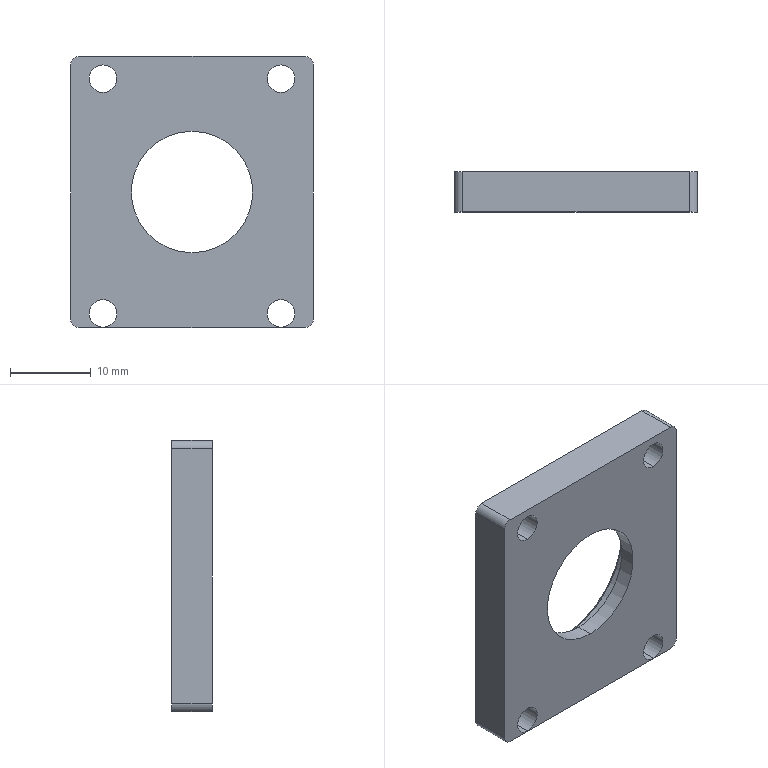Component | SolidWorks | FocusingLensHolder-1 | 1 solid | 25 faces | box 30 x 5 x 33.5 mm | volume 3535 mm3 | cylinder 16 | plane 7 | cone 2 | commonest cylinder face diameters 3.4 x8 2 x4 20 x2 15 x2
build123d program:
from build123d import *

# Parameters (mm, degrees)
SKETCH1_W           = 30
SKETCH1_H           = 33.5
SKETCH1_R           = 1.7
BOSS_EXTRUDE1_DEPTH = 5
SKETCH2_R           = 7.5
CUT_EXTRUDE1_DEPTH  = 6
SKETCH3_R           = 10
CUT_EXTRUDE2_DEPTH  = 3
CHAMFER1_SIZE       = 0.5
FILLET1_R           = 1


with BuildPart() as part:
    # Sketch1 → Boss-Extrude1 (new body)
    with BuildSketch(Plane(origin=(0, 0, 0), x_dir=(1, 0, 0), z_dir=(0, 1, 0))):
        Rectangle(SKETCH1_W, SKETCH1_H)
        with Locations(Location((-11, -14, 0), (0, 0, 270))):
            Circle(SKETCH1_R, mode=Mode.SUBTRACT)
        with Locations(Location((11, -14, 0), (0, 0, 90))):
            Circle(SKETCH1_R, mode=Mode.SUBTRACT)
        with Locations(Location((-11, 15, 0), (0, 0, 270))):
            Circle(SKETCH1_R, mode=Mode.SUBTRACT)
        with Locations(Location((11, 15, 0), (0, 0, 270))):
            Circle(SKETCH1_R, mode=Mode.SUBTRACT)
    extrude(amount=BOSS_EXTRUDE1_DEPTH)

    # Sketch2 → Cut-Extrude1 (cut)
    with BuildSketch(Plane(origin=(0, 5, 0), x_dir=(1, 0, 0), z_dir=(0, 1, 0))):
        with Locations(Location((0, 0, 0), (0, 0, 270))):
            Circle(SKETCH2_R)
    extrude(amount=-CUT_EXTRUDE1_DEPTH, mode=Mode.SUBTRACT)

    # Sketch3 → Cut-Extrude2 (cut)
    with BuildSketch(Plane(origin=(0, 5, 0), x_dir=(1, 0, 0), z_dir=(0, 1, 0))):
        with Locations(Location((0, 0, 0), (0, 0, 270))):
            Circle(SKETCH3_R)
    extrude(amount=-CUT_EXTRUDE2_DEPTH, mode=Mode.SUBTRACT)

    # Chamfer1
    chamfer1_edges = [part.edges().sort_by_distance(p)[0] for p in [
        (0, 5, -10),
    ]]
    chamfer(chamfer1_edges, length=CHAMFER1_SIZE)

    # Fillet1
    fillet1_edges = [part.edges().sort_by_distance(p)[0] for p in [
        (15, 2.5, 16.75),
        (-15, 2.5, 16.75),
        (-15, 2.5, -16.75),
        (15, 2.5, -16.75),
    ]]
    fillet(fillet1_edges, radius=FILLET1_R)


solid = part.part

# Placed as in the assembly
solid = solid.moved(Location((-5.981, 10.506, 205.812), (0, 0, 0)))
STEP:
#1=COLOUR_RGB('',0.7922,0.8196,0.9333);
#2=FILL_AREA_STYLE_COLOUR('',#1);
#3=FILL_AREA_STYLE('',(#2));
#4=SURFACE_STYLE_FILL_AREA(#3);
#5=SURFACE_SIDE_STYLE('',(#4));
#6=SURFACE_STYLE_USAGE(.BOTH.,#5);
#7=PRESENTATION_STYLE_ASSIGNMENT((#6));
#8=CARTESIAN_POINT('',(-0.2355,0.5908,7.709));
#9=VERTEX_POINT('',#8);
#10=CARTESIAN_POINT('',(-0.2355,0.5908,8.497));
#11=VERTEX_POINT('',#10);
#12=CARTESIAN_POINT('',(-0.2355,0.5908,8.103));
#13=DIRECTION('',(0.,1.,0.));
#14=DIRECTION('',(0.,0.,1.));
#15=AXIS2_PLACEMENT_3D('',#12,#13,#14);
#16=CIRCLE('',#15,0.3937);
#17=EDGE_CURVE('',#9,#11,#16,.T.);
#18=ORIENTED_EDGE('',*,*,#17,.F.);
#19=CARTESIAN_POINT('',(-0.2355,0.6105,7.689));
#20=VERTEX_POINT('',#19);
#21=CARTESIAN_POINT('',(-0.2355,0.5908,7.709));
#22=DIRECTION('',(0.,0.7071,-0.7071));
#23=VECTOR('',#22,39.37);
#24=LINE('',#21,#23);
#25=EDGE_CURVE('',#9,#20,#24,.T.);
#26=ORIENTED_EDGE('',*,*,#25,.T.);
#27=CARTESIAN_POINT('',(-0.2355,0.6105,8.516));
#28=VERTEX_POINT('',#27);
#29=CARTESIAN_POINT('',(-0.2355,0.6105,8.103));
#30=DIRECTION('',(0.,-1.,0.));
#31=DIRECTION('',(0.,0.,1.));
#32=AXIS2_PLACEMENT_3D('',#29,#30,#31);
#33=CIRCLE('',#32,0.4134);
#34=EDGE_CURVE('',#28,#20,#33,.T.);
#35=ORIENTED_EDGE('',*,*,#34,.F.);
#36=CARTESIAN_POINT('',(-0.2355,0.5908,8.497));
#37=DIRECTION('',(0.,0.7071,0.7071));
#38=VECTOR('',#37,39.37);
#39=LINE('',#36,#38);
#40=EDGE_CURVE('',#11,#28,#39,.T.);
#41=ORIENTED_EDGE('',*,*,#40,.F.);
#42=EDGE_LOOP('',(#18,#26,#35,#41));
#43=FACE_OUTER_BOUND('',#42,.T.);
#44=CARTESIAN_POINT('',(-0.2355,0.5908,8.103));
#45=DIRECTION('',(0.,1.,0.));
#46=DIRECTION('',(0.,0.,1.));
#47=AXIS2_PLACEMENT_3D('',#44,#45,#46);
#48=CONICAL_SURFACE('',#47,0.3937,0.7854);
#49=ADVANCED_FACE('',(#43),#48,.F.);
#50=CARTESIAN_POINT('',(-0.2355,0.4924,7.709));
#51=VERTEX_POINT('',#50);
#52=CARTESIAN_POINT('',(-0.2355,0.4924,8.497));
#53=VERTEX_POINT('',#52);
#54=CARTESIAN_POINT('',(-0.2355,0.4924,8.103));
#55=DIRECTION('',(0.,1.,0.));
#56=DIRECTION('',(0.,0.,1.));
#57=AXIS2_PLACEMENT_3D('',#54,#55,#56);
#58=CIRCLE('',#57,0.3937);
#59=EDGE_CURVE('',#51,#53,#58,.T.);
#60=ORIENTED_EDGE('',*,*,#59,.F.);
#61=CARTESIAN_POINT('',(-0.2355,0.4924,7.709));
#62=DIRECTION('',(0.,1.,0.));
#63=VECTOR('',#62,39.37);
#64=LINE('',#61,#63);
#65=EDGE_CURVE('',#51,#9,#64,.T.);
#66=ORIENTED_EDGE('',*,*,#65,.T.);
#67=ORIENTED_EDGE('',*,*,#17,.T.);
#68=CARTESIAN_POINT('',(-0.2355,0.4924,8.497));
#69=DIRECTION('',(0.,1.,0.));
#70=VECTOR('',#69,39.37);
#71=LINE('',#68,#70);
#72=EDGE_CURVE('',#53,#11,#71,.T.);
#73=ORIENTED_EDGE('',*,*,#72,.F.);
#74=EDGE_LOOP('',(#60,#66,#67,#73));
#75=FACE_OUTER_BOUND('',#74,.T.);
#76=CARTESIAN_POINT('',(-0.2355,0.4924,8.103));
#77=DIRECTION('',(0.,1.,0.));
#78=DIRECTION('',(0.,0.,1.));
#79=AXIS2_PLACEMENT_3D('',#76,#77,#78);
#80=CYLINDRICAL_SURFACE('',#79,0.3937);
#81=ADVANCED_FACE('',(#75),#80,.F.);
#82=CARTESIAN_POINT('',(0.1976,0.6105,7.445));
#83=VERTEX_POINT('',#82);
#84=CARTESIAN_POINT('',(0.1976,0.6105,7.579));
#85=VERTEX_POINT('',#84);
#86=CARTESIAN_POINT('',(0.1976,0.6105,7.512));
#87=DIRECTION('',(0.,1.,0.));
#88=DIRECTION('',(0.,0.,1.));
#89=AXIS2_PLACEMENT_3D('',#86,#87,#88);
#90=CIRCLE('',#89,0.06693);
#91=EDGE_CURVE('',#83,#85,#90,.T.);
#92=ORIENTED_EDGE('',*,*,#91,.T.);
#93=CARTESIAN_POINT('',(0.1976,0.4136,7.579));
#94=VERTEX_POINT('',#93);
#95=CARTESIAN_POINT('',(0.1976,0.6105,7.579));
#96=DIRECTION('',(0.,-1.,0.));
#97=VECTOR('',#96,39.37);
#98=LINE('',#95,#97);
#99=EDGE_CURVE('',#85,#94,#98,.T.);
#100=ORIENTED_EDGE('',*,*,#99,.T.);
#101=CARTESIAN_POINT('',(0.1976,0.4136,7.445));
#102=VERTEX_POINT('',#101);
#103=CARTESIAN_POINT('',(0.1976,0.4136,7.512));
#104=DIRECTION('',(0.,1.,0.));
#105=DIRECTION('',(0.,0.,1.));
#106=AXIS2_PLACEMENT_3D('',#103,#104,#105);
#107=CIRCLE('',#106,0.06693);
#108=EDGE_CURVE('',#102,#94,#107,.T.);
#109=ORIENTED_EDGE('',*,*,#108,.F.);
#110=CARTESIAN_POINT('',(0.1976,0.6105,7.445));
#111=DIRECTION('',(0.,-1.,0.));
#112=VECTOR('',#111,39.37);
#113=LINE('',#110,#112);
#114=EDGE_CURVE('',#83,#102,#113,.T.);
#115=ORIENTED_EDGE('',*,*,#114,.F.);
#116=EDGE_LOOP('',(#92,#100,#109,#115));
#117=FACE_OUTER_BOUND('',#116,.T.);
#118=CARTESIAN_POINT('',(0.1976,0.6105,7.512));
#119=DIRECTION('',(0.,-1.,0.));
#120=DIRECTION('',(0.,0.,-1.));
#121=AXIS2_PLACEMENT_3D('',#118,#119,#120);
#122=CYLINDRICAL_SURFACE('',#121,0.06693);
#123=ADVANCED_FACE('',(#117),#122,.F.);
#124=CARTESIAN_POINT('',(-0.6685,0.6105,7.445));
#125=VERTEX_POINT('',#124);
#126=CARTESIAN_POINT('',(-0.6685,0.6105,7.579));
#127=VERTEX_POINT('',#126);
#128=CARTESIAN_POINT('',(-0.6685,0.6105,7.512));
#129=DIRECTION('',(0.,1.,0.));
#130=DIRECTION('',(0.,0.,1.));
#131=AXIS2_PLACEMENT_3D('',#128,#129,#130);
#132=CIRCLE('',#131,0.06693);
#133=EDGE_CURVE('',#125,#127,#132,.T.);
#134=ORIENTED_EDGE('',*,*,#133,.T.);
#135=CARTESIAN_POINT('',(-0.6685,0.4136,7.579));
#136=VERTEX_POINT('',#135);
#137=CARTESIAN_POINT('',(-0.6685,0.6105,7.579));
#138=DIRECTION('',(0.,-1.,0.));
#139=VECTOR('',#138,39.37);
#140=LINE('',#137,#139);
#141=EDGE_CURVE('',#127,#136,#140,.T.);
#142=ORIENTED_EDGE('',*,*,#141,.T.);
#143=CARTESIAN_POINT('',(-0.6685,0.4136,7.445));
#144=VERTEX_POINT('',#143);
#145=CARTESIAN_POINT('',(-0.6685,0.4136,7.512));
#146=DIRECTION('',(0.,1.,0.));
#147=DIRECTION('',(0.,0.,1.));
#148=AXIS2_PLACEMENT_3D('',#145,#146,#147);
#149=CIRCLE('',#148,0.06693);
#150=EDGE_CURVE('',#144,#136,#149,.T.);
#151=ORIENTED_EDGE('',*,*,#150,.F.);
#152=CARTESIAN_POINT('',(-0.6685,0.6105,7.445));
#153=DIRECTION('',(0.,-1.,0.));
#154=VECTOR('',#153,39.37);
#155=LINE('',#152,#154);
#156=EDGE_CURVE('',#125,#144,#155,.T.);
#157=ORIENTED_EDGE('',*,*,#156,.F.);
#158=EDGE_LOOP('',(#134,#142,#151,#157));
#159=FACE_OUTER_BOUND('',#158,.T.);
#160=CARTESIAN_POINT('',(-0.6685,0.6105,7.512));
#161=DIRECTION('',(0.,-1.,0.));
#162=DIRECTION('',(0.,0.,-1.));
#163=AXIS2_PLACEMENT_3D('',#160,#161,#162);
#164=CYLINDRICAL_SURFACE('',#163,0.06693);
#165=ADVANCED_FACE('',(#159),#164,.F.);
#166=CARTESIAN_POINT('',(0.1976,0.6105,8.587));
#167=VERTEX_POINT('',#166);
#168=CARTESIAN_POINT('',(0.1976,0.6105,8.721));
#169=VERTEX_POINT('',#168);
#170=CARTESIAN_POINT('',(0.1976,0.6105,8.654));
#171=DIRECTION('',(0.,1.,0.));
#172=DIRECTION('',(0.,0.,-1.));
#173=AXIS2_PLACEMENT_3D('',#170,#171,#172);
#174=CIRCLE('',#173,0.06693);
#175=EDGE_CURVE('',#167,#169,#174,.T.);
#176=ORIENTED_EDGE('',*,*,#175,.T.);
#177=CARTESIAN_POINT('',(0.1976,0.4136,8.721));
#178=VERTEX_POINT('',#177);
#179=CARTESIAN_POINT('',(0.1976,0.6105,8.721));
#180=DIRECTION('',(0.,-1.,0.));
#181=VECTOR('',#180,39.37);
#182=LINE('',#179,#181);
#183=EDGE_CURVE('',#169,#178,#182,.T.);
#184=ORIENTED_EDGE('',*,*,#183,.T.);
#185=CARTESIAN_POINT('',(0.1976,0.4136,8.587));
#186=VERTEX_POINT('',#185);
#187=CARTESIAN_POINT('',(0.1976,0.4136,8.654));
#188=DIRECTION('',(0.,1.,0.));
#189=DIRECTION('',(0.,0.,-1.));
#190=AXIS2_PLACEMENT_3D('',#187,#188,#189);
#191=CIRCLE('',#190,0.06693);
#192=EDGE_CURVE('',#186,#178,#191,.T.);
#193=ORIENTED_EDGE('',*,*,#192,.F.);
#194=CARTESIAN_POINT('',(0.1976,0.6105,8.587));
#195=DIRECTION('',(0.,-1.,0.));
#196=VECTOR('',#195,39.37);
#197=LINE('',#194,#196);
#198=EDGE_CURVE('',#167,#186,#197,.T.);
#199=ORIENTED_EDGE('',*,*,#198,.F.);
#200=EDGE_LOOP('',(#176,#184,#193,#199));
#201=FACE_OUTER_BOUND('',#200,.T.);
#202=CARTESIAN_POINT('',(0.1976,0.6105,8.654));
#203=DIRECTION('',(0.,-1.,0.));
#204=DIRECTION('',(0.,0.,-1.));
#205=AXIS2_PLACEMENT_3D('',#202,#203,#204);
#206=CYLINDRICAL_SURFACE('',#205,0.06693);
#207=ADVANCED_FACE('',(#201),#206,.F.);
#208=CARTESIAN_POINT('',(-0.6685,0.6105,8.587));
#209=VERTEX_POINT('',#208);
#210=CARTESIAN_POINT('',(-0.6685,0.6105,8.721));
#211=VERTEX_POINT('',#210);
#212=CARTESIAN_POINT('',(-0.6685,0.6105,8.654));
#213=DIRECTION('',(0.,1.,0.));
#214=DIRECTION('',(0.,0.,1.));
#215=AXIS2_PLACEMENT_3D('',#212,#213,#214);
#216=CIRCLE('',#215,0.06693);
#217=EDGE_CURVE('',#209,#211,#216,.T.);
#218=ORIENTED_EDGE('',*,*,#217,.T.);
#219=CARTESIAN_POINT('',(-0.6685,0.4136,8.721));
#220=VERTEX_POINT('',#219);
#221=CARTESIAN_POINT('',(-0.6685,0.6105,8.721));
#222=DIRECTION('',(0.,-1.,0.));
#223=VECTOR('',#222,39.37);
#224=LINE('',#221,#223);
#225=EDGE_CURVE('',#211,#220,#224,.T.);
#226=ORIENTED_EDGE('',*,*,#225,.T.);
#227=CARTESIAN_POINT('',(-0.6685,0.4136,8.587));
#228=VERTEX_POINT('',#227);
#229=CARTESIAN_POINT('',(-0.6685,0.4136,8.654));
#230=DIRECTION('',(0.,1.,0.));
#231=DIRECTION('',(0.,0.,1.));
#232=AXIS2_PLACEMENT_3D('',#229,#230,#231);
#233=CIRCLE('',#232,0.06693);
#234=EDGE_CURVE('',#228,#220,#233,.T.);
#235=ORIENTED_EDGE('',*,*,#234,.F.);
#236=CARTESIAN_POINT('',(-0.6685,0.6105,8.587));
#237=DIRECTION('',(0.,-1.,0.));
#238=VECTOR('',#237,39.37);
#239=LINE('',#236,#238);
#240=EDGE_CURVE('',#209,#228,#239,.T.);
#241=ORIENTED_EDGE('',*,*,#240,.F.);
#242=EDGE_LOOP('',(#218,#226,#235,#241));
#243=FACE_OUTER_BOUND('',#242,.T.);
#244=CARTESIAN_POINT('',(-0.6685,0.6105,8.654));
#245=DIRECTION('',(0.,-1.,0.));
#246=DIRECTION('',(0.,0.,-1.));
#247=AXIS2_PLACEMENT_3D('',#244,#245,#246);
#248=CYLINDRICAL_SURFACE('',#247,0.06693);
#249=ADVANCED_FACE('',(#243),#248,.F.);
#250=CARTESIAN_POINT('',(-0.2355,0.4136,7.808));
#251=VERTEX_POINT('',#250);
#252=CARTESIAN_POINT('',(-0.2355,0.4136,8.398));
#253=VERTEX_POINT('',#252);
#254=CARTESIAN_POINT('',(-0.2355,0.4136,8.103));
#255=DIRECTION('',(0.,1.,0.));
#256=DIRECTION('',(0.,0.,1.));
#257=AXIS2_PLACEMENT_3D('',#254,#255,#256);
#258=CIRCLE('',#257,0.2953);
#259=EDGE_CURVE('',#251,#253,#258,.T.);
#260=ORIENTED_EDGE('',*,*,#259,.F.);
#261=CARTESIAN_POINT('',(-0.2355,0.4924,7.808));
#262=VERTEX_POINT('',#261);
#263=CARTESIAN_POINT('',(-0.2355,0.3743,7.808));
#264=DIRECTION('',(0.,1.,0.));
#265=VECTOR('',#264,39.37);
#266=LINE('',#263,#265);
#267=EDGE_CURVE('',#251,#262,#266,.T.);
#268=ORIENTED_EDGE('',*,*,#267,.T.);
#269=CARTESIAN_POINT('',(-0.2355,0.4924,8.398));
#270=VERTEX_POINT('',#269);
#271=CARTESIAN_POINT('',(-0.2355,0.4924,8.103));
#272=DIRECTION('',(0.,-1.,0.));
#273=DIRECTION('',(0.,0.,1.));
#274=AXIS2_PLACEMENT_3D('',#271,#272,#273);
#275=CIRCLE('',#274,0.2953);
#276=EDGE_CURVE('',#270,#262,#275,.T.);
#277=ORIENTED_EDGE('',*,*,#276,.F.);
#278=CARTESIAN_POINT('',(-0.2355,0.3743,8.398));
#279=DIRECTION('',(0.,1.,0.));
#280=VECTOR('',#279,39.37);
#281=LINE('',#278,#280);
#282=EDGE_CURVE('',#253,#270,#281,.T.);
#283=ORIENTED_EDGE('',*,*,#282,.F.);
#284=EDGE_LOOP('',(#260,#268,#277,#283));
#285=FACE_OUTER_BOUND('',#284,.T.);
#286=CARTESIAN_POINT('',(-0.2355,0.3743,8.103));
#287=DIRECTION('',(0.,1.,0.));
#288=DIRECTION('',(0.,0.,1.));
#289=AXIS2_PLACEMENT_3D('',#286,#287,#288);
#290=CYLINDRICAL_SURFACE('',#289,0.2953);
#291=ADVANCED_FACE('',(#285),#290,.F.);
#292=ORIENTED_EDGE('',*,*,#267,.F.);
#293=CARTESIAN_POINT('',(-0.2355,0.4136,8.103));
#294=DIRECTION('',(0.,1.,0.));
#295=DIRECTION('',(0.,0.,1.));
#296=AXIS2_PLACEMENT_3D('',#293,#294,#295);
#297=CIRCLE('',#296,0.2953);
#298=EDGE_CURVE('',#253,#251,#297,.T.);
#299=ORIENTED_EDGE('',*,*,#298,.F.);
#300=ORIENTED_EDGE('',*,*,#282,.T.);
#301=CARTESIAN_POINT('',(-0.2355,0.4924,8.103));
#302=DIRECTION('',(0.,-1.,0.));
#303=DIRECTION('',(0.,0.,1.));
#304=AXIS2_PLACEMENT_3D('',#301,#302,#303);
#305=CIRCLE('',#304,0.2953);
#306=EDGE_CURVE('',#262,#270,#305,.T.);
#307=ORIENTED_EDGE('',*,*,#306,.F.);
#308=EDGE_LOOP('',(#292,#299,#300,#307));
#309=FACE_OUTER_BOUND('',#308,.T.);
#310=CARTESIAN_POINT('',(-0.2355,0.3743,8.103));
#311=DIRECTION('',(0.,1.,0.));
#312=DIRECTION('',(0.,0.,1.));
#313=AXIS2_PLACEMENT_3D('',#310,#311,#312);
#314=CYLINDRICAL_SURFACE('',#313,0.2953);
#315=ADVANCED_FACE('',(#309),#314,.F.);
#316=ORIENTED_EDGE('',*,*,#34,.T.);
#317=CARTESIAN_POINT('',(-0.2355,0.6105,8.103));
#318=DIRECTION('',(0.,-1.,0.));
#319=DIRECTION('',(0.,0.,1.));
#320=AXIS2_PLACEMENT_3D('',#317,#318,#319);
#321=CIRCLE('',#320,0.4134);
#322=EDGE_CURVE('',#20,#28,#321,.T.);
#323=ORIENTED_EDGE('',*,*,#322,.T.);
#324=EDGE_LOOP('',(#316,#323));
#325=FACE_BOUND('',#324,.T.);
#326=ORIENTED_EDGE('',*,*,#133,.F.);
#327=CARTESIAN_POINT('',(-0.6685,0.6105,7.512));
#328=DIRECTION('',(0.,1.,0.));
#329=DIRECTION('',(0.,0.,1.));
#330=AXIS2_PLACEMENT_3D('',#327,#328,#329);
#331=CIRCLE('',#330,0.06693);
#332=EDGE_CURVE('',#127,#125,#331,.T.);
#333=ORIENTED_EDGE('',*,*,#332,.F.);
#334=EDGE_LOOP('',(#326,#333));
#335=FACE_BOUND('',#334,.T.);
#336=ORIENTED_EDGE('',*,*,#217,.F.);
#337=CARTESIAN_POINT('',(-0.6685,0.6105,8.654));
#338=DIRECTION('',(0.,1.,0.));
#339=DIRECTION('',(0.,0.,1.));
#340=AXIS2_PLACEMENT_3D('',#337,#338,#339);
#341=CIRCLE('',#340,0.06693);
#342=EDGE_CURVE('',#211,#209,#341,.T.);
#343=ORIENTED_EDGE('',*,*,#342,.F.);
#344=EDGE_LOOP('',(#336,#343));
#345=FACE_BOUND('',#344,.T.);
#346=CARTESIAN_POINT('',(-0.826,0.6105,7.483));
#347=VERTEX_POINT('',#346);
#348=CARTESIAN_POINT('',(-0.826,0.6105,8.723));
#349=VERTEX_POINT('',#348);
#350=CARTESIAN_POINT('',(-0.826,0.6105,7.443));
#351=DIRECTION('',(-0.,0.,1.));
#352=VECTOR('',#351,39.37);
#353=LINE('',#350,#352);
#354=EDGE_CURVE('',#347,#349,#353,.T.);
#355=ORIENTED_EDGE('',*,*,#354,.T.);
#356=CARTESIAN_POINT('',(-0.7866,0.6105,8.762));
#357=VERTEX_POINT('',#356);
#358=CARTESIAN_POINT('',(-0.7866,0.6105,8.723));
#359=DIRECTION('',(0.,1.,0.));
#360=DIRECTION('',(0.,0.,1.));
#361=AXIS2_PLACEMENT_3D('',#358,#359,#360);
#362=CIRCLE('',#361,0.03937);
#363=EDGE_CURVE('',#349,#357,#362,.T.);
#364=ORIENTED_EDGE('',*,*,#363,.T.);
#365=CARTESIAN_POINT('',(0.3157,0.6105,8.762));
#366=VERTEX_POINT('',#365);
#367=CARTESIAN_POINT('',(-0.826,0.6105,8.762));
#368=DIRECTION('',(1.,0.,0.));
#369=VECTOR('',#368,39.37);
#370=LINE('',#367,#369);
#371=EDGE_CURVE('',#357,#366,#370,.T.);
#372=ORIENTED_EDGE('',*,*,#371,.T.);
#373=CARTESIAN_POINT('',(0.3551,0.6105,8.723));
#374=VERTEX_POINT('',#373);
#375=CARTESIAN_POINT('',(0.3157,0.6105,8.723));
#376=DIRECTION('',(0.,1.,0.));
#377=DIRECTION('',(0.,0.,1.));
#378=AXIS2_PLACEMENT_3D('',#375,#376,#377);
#379=CIRCLE('',#378,0.03937);
#380=EDGE_CURVE('',#366,#374,#379,.T.);
#381=ORIENTED_EDGE('',*,*,#380,.T.);
#382=CARTESIAN_POINT('',(0.3551,0.6105,7.483));
#383=VERTEX_POINT('',#382);
#384=CARTESIAN_POINT('',(0.3551,0.6105,7.443));
#385=DIRECTION('',(0.,0.,-1.));
#386=VECTOR('',#385,39.37);
#387=LINE('',#384,#386);
#388=EDGE_CURVE('',#374,#383,#387,.T.);
#389=ORIENTED_EDGE('',*,*,#388,.T.);
#390=CARTESIAN_POINT('',(0.3157,0.6105,7.443));
#391=VERTEX_POINT('',#390);
#392=CARTESIAN_POINT('',(0.3157,0.6105,7.483));
#393=DIRECTION('',(0.,1.,0.));
#394=DIRECTION('',(0.,0.,1.));
#395=AXIS2_PLACEMENT_3D('',#392,#393,#394);
#396=CIRCLE('',#395,0.03937);
#397=EDGE_CURVE('',#383,#391,#396,.T.);
#398=ORIENTED_EDGE('',*,*,#397,.T.);
#399=CARTESIAN_POINT('',(-0.7866,0.6105,7.443));
#400=VERTEX_POINT('',#399);
#401=CARTESIAN_POINT('',(-0.826,0.6105,7.443));
#402=DIRECTION('',(-1.,0.,-0.));
#403=VECTOR('',#402,39.37);
#404=LINE('',#401,#403);
#405=EDGE_CURVE('',#391,#400,#404,.T.);
#406=ORIENTED_EDGE('',*,*,#405,.T.);
#407=CARTESIAN_POINT('',(-0.7866,0.6105,7.483));
#408=DIRECTION('',(0.,1.,0.));
#409=DIRECTION('',(0.,0.,1.));
#410=AXIS2_PLACEMENT_3D('',#407,#408,#409);
#411=CIRCLE('',#410,0.03937);
#412=EDGE_CURVE('',#400,#347,#411,.T.);
#413=ORIENTED_EDGE('',*,*,#412,.T.);
#414=EDGE_LOOP('',(#355,#364,#372,#381,#389,#398,#406,#413));
#415=FACE_OUTER_BOUND('',#414,.T.);
#416=ORIENTED_EDGE('',*,*,#175,.F.);
#417=CARTESIAN_POINT('',(0.1976,0.6105,8.654));
#418=DIRECTION('',(0.,1.,0.));
#419=DIRECTION('',(0.,0.,-1.));
#420=AXIS2_PLACEMENT_3D('',#417,#418,#419);
#421=CIRCLE('',#420,0.06693);
#422=EDGE_CURVE('',#169,#167,#421,.T.);
#423=ORIENTED_EDGE('',*,*,#422,.F.);
#424=EDGE_LOOP('',(#416,#423));
#425=FACE_BOUND('',#424,.T.);
#426=ORIENTED_EDGE('',*,*,#91,.F.);
#427=CARTESIAN_POINT('',(0.1976,0.6105,7.512));
#428=DIRECTION('',(0.,1.,0.));
#429=DIRECTION('',(0.,0.,1.));
#430=AXIS2_PLACEMENT_3D('',#427,#428,#429);
#431=CIRCLE('',#430,0.06693);
#432=EDGE_CURVE('',#85,#83,#431,.T.);
#433=ORIENTED_EDGE('',*,*,#432,.F.);
#434=EDGE_LOOP('',(#426,#433));
#435=FACE_BOUND('',#434,.T.);
#436=CARTESIAN_POINT('',(-0.2355,0.6105,8.103));
#437=DIRECTION('',(0.,1.,0.));
#438=DIRECTION('',(0.,0.,1.));
#439=AXIS2_PLACEMENT_3D('',#436,#437,#438);
#440=PLANE('',#439);
#441=ADVANCED_FACE('',(#325,#335,#345,#415,#425,#435),#440,.T.);
#442=ORIENTED_EDGE('',*,*,#298,.T.);
#443=ORIENTED_EDGE('',*,*,#259,.T.);
#444=EDGE_LOOP('',(#442,#443));
#445=FACE_BOUND('',#444,.T.);
#446=CARTESIAN_POINT('',(-0.7866,0.4136,8.762));
#447=VERTEX_POINT('',#446);
#448=CARTESIAN_POINT('',(0.3157,0.4136,8.762));
#449=VERTEX_POINT('',#448);
#450=CARTESIAN_POINT('',(-0.826,0.4136,8.762));
#451=DIRECTION('',(1.,0.,0.));
#452=VECTOR('',#451,39.37);
#453=LINE('',#450,#452);
#454=EDGE_CURVE('',#447,#449,#453,.T.);
#455=ORIENTED_EDGE('',*,*,#454,.F.);
#456=CARTESIAN_POINT('',(-0.826,0.4136,8.723));
#457=VERTEX_POINT('',#456);
#458=CARTESIAN_POINT('',(-0.7866,0.4136,8.723));
#459=DIRECTION('',(0.,-1.,0.));
#460=DIRECTION('',(0.,0.,1.));
#461=AXIS2_PLACEMENT_3D('',#458,#459,#460);
#462=CIRCLE('',#461,0.03937);
#463=EDGE_CURVE('',#447,#457,#462,.T.);
#464=ORIENTED_EDGE('',*,*,#463,.T.);
#465=CARTESIAN_POINT('',(-0.826,0.4136,7.483));
#466=VERTEX_POINT('',#465);
#467=CARTESIAN_POINT('',(-0.826,0.4136,7.443));
#468=DIRECTION('',(-0.,0.,1.));
#469=VECTOR('',#468,39.37);
#470=LINE('',#467,#469);
#471=EDGE_CURVE('',#466,#457,#470,.T.);
#472=ORIENTED_EDGE('',*,*,#471,.F.);
#473=CARTESIAN_POINT('',(-0.7866,0.4136,7.443));
#474=VERTEX_POINT('',#473);
#475=CARTESIAN_POINT('',(-0.7866,0.4136,7.483));
#476=DIRECTION('',(0.,-1.,0.));
#477=DIRECTION('',(0.,0.,1.));
#478=AXIS2_PLACEMENT_3D('',#475,#476,#477);
#479=CIRCLE('',#478,0.03937);
#480=EDGE_CURVE('',#466,#474,#479,.T.);
#481=ORIENTED_EDGE('',*,*,#480,.T.);
#482=CARTESIAN_POINT('',(0.3157,0.4136,7.443));
#483=VERTEX_POINT('',#482);
#484=CARTESIAN_POINT('',(-0.826,0.4136,7.443));
#485=DIRECTION('',(-1.,0.,-0.));
#486=VECTOR('',#485,39.37);
#487=LINE('',#484,#486);
#488=EDGE_CURVE('',#483,#474,#487,.T.);
#489=ORIENTED_EDGE('',*,*,#488,.F.);
#490=CARTESIAN_POINT('',(0.3551,0.4136,7.483));
#491=VERTEX_POINT('',#490);
#492=CARTESIAN_POINT('',(0.3157,0.4136,7.483));
#493=DIRECTION('',(0.,-1.,0.));
#494=DIRECTION('',(0.,0.,1.));
#495=AXIS2_PLACEMENT_3D('',#492,#493,#494);
#496=CIRCLE('',#495,0.03937);
#497=EDGE_CURVE('',#483,#491,#496,.T.);
#498=ORIENTED_EDGE('',*,*,#497,.T.);
#499=CARTESIAN_POINT('',(0.3551,0.4136,8.723));
#500=VERTEX_POINT('',#499);
#501=CARTESIAN_POINT('',(0.3551,0.4136,7.443));
#502=DIRECTION('',(0.,0.,-1.));
#503=VECTOR('',#502,39.37);
#504=LINE('',#501,#503);
#505=EDGE_CURVE('',#500,#491,#504,.T.);
#506=ORIENTED_EDGE('',*,*,#505,.F.);
#507=CARTESIAN_POINT('',(0.3157,0.4136,8.723));
#508=DIRECTION('',(0.,-1.,0.));
#509=DIRECTION('',(0.,0.,1.));
#510=AXIS2_PLACEMENT_3D('',#507,#508,#509);
#511=CIRCLE('',#510,0.03937);
#512=EDGE_CURVE('',#500,#449,#511,.T.);
#513=ORIENTED_EDGE('',*,*,#512,.T.);
#514=EDGE_LOOP('',(#455,#464,#472,#481,#489,#498,#506,#513));
#515=FACE_OUTER_BOUND('',#514,.T.);
#516=ORIENTED_EDGE('',*,*,#234,.T.);
#517=CARTESIAN_POINT('',(-0.6685,0.4136,8.654));
#518=DIRECTION('',(0.,1.,0.));
#519=DIRECTION('',(0.,0.,1.));
#520=AXIS2_PLACEMENT_3D('',#517,#518,#519);
#521=CIRCLE('',#520,0.06693);
#522=EDGE_CURVE('',#220,#228,#521,.T.);
#523=ORIENTED_EDGE('',*,*,#522,.T.);
#524=EDGE_LOOP('',(#516,#523));
#525=FACE_BOUND('',#524,.T.);
#526=ORIENTED_EDGE('',*,*,#192,.T.);
#527=CARTESIAN_POINT('',(0.1976,0.4136,8.654));
#528=DIRECTION('',(0.,1.,0.));
#529=DIRECTION('',(0.,0.,-1.));
#530=AXIS2_PLACEMENT_3D('',#527,#528,#529);
#531=CIRCLE('',#530,0.06693);
#532=EDGE_CURVE('',#178,#186,#531,.T.);
#533=ORIENTED_EDGE('',*,*,#532,.T.);
#534=EDGE_LOOP('',(#526,#533));
#535=FACE_BOUND('',#534,.T.);
#536=ORIENTED_EDGE('',*,*,#150,.T.);
#537=CARTESIAN_POINT('',(-0.6685,0.4136,7.512));
#538=DIRECTION('',(0.,1.,0.));
#539=DIRECTION('',(0.,0.,1.));
#540=AXIS2_PLACEMENT_3D('',#537,#538,#539);
#541=CIRCLE('',#540,0.06693);
#542=EDGE_CURVE('',#136,#144,#541,.T.);
#543=ORIENTED_EDGE('',*,*,#542,.T.);
#544=EDGE_LOOP('',(#536,#543));
#545=FACE_BOUND('',#544,.T.);
#546=ORIENTED_EDGE('',*,*,#108,.T.);
#547=CARTESIAN_POINT('',(0.1976,0.4136,7.512));
#548=DIRECTION('',(0.,1.,0.));
#549=DIRECTION('',(0.,0.,1.));
#550=AXIS2_PLACEMENT_3D('',#547,#548,#549);
#551=CIRCLE('',#550,0.06693);
#552=EDGE_CURVE('',#94,#102,#551,.T.);
#553=ORIENTED_EDGE('',*,*,#552,.T.);
#554=EDGE_LOOP('',(#546,#553));
#555=FACE_BOUND('',#554,.T.);
#556=CARTESIAN_POINT('',(-0.2355,0.4136,8.103));
#557=DIRECTION('',(0.,1.,0.));
#558=DIRECTION('',(0.,0.,1.));
#559=AXIS2_PLACEMENT_3D('',#556,#557,#558);
#560=PLANE('',#559);
#561=ADVANCED_FACE('',(#445,#515,#525,#535,#545,#555),#560,.F.);
#562=ORIENTED_EDGE('',*,*,#505,.T.);
#563=CARTESIAN_POINT('',(0.3551,0.6105,7.483));
#564=DIRECTION('',(0.,1.,0.));
#565=VECTOR('',#564,39.37);
#566=LINE('',#563,#565);
#567=EDGE_CURVE('',#491,#383,#566,.T.);
#568=ORIENTED_EDGE('',*,*,#567,.T.);
#569=ORIENTED_EDGE('',*,*,#388,.F.);
#570=CARTESIAN_POINT('',(0.3551,0.6105,8.723));
#571=DIRECTION('',(0.,-1.,0.));
#572=VECTOR('',#571,39.37);
#573=LINE('',#570,#572);
#574=EDGE_CURVE('',#374,#500,#573,.T.);
#575=ORIENTED_EDGE('',*,*,#574,.T.);
#576=EDGE_LOOP('',(#562,#568,#569,#575));
#577=FACE_OUTER_BOUND('',#576,.T.);
#578=CARTESIAN_POINT('',(0.3551,0.6105,7.443));
#579=DIRECTION('',(-1.,0.,-0.));
#580=DIRECTION('',(-0.,0.,1.));
#581=AXIS2_PLACEMENT_3D('',#578,#579,#580);
#582=PLANE('',#581);
#583=ADVANCED_FACE('',(#577),#582,.F.);
#584=ORIENTED_EDGE('',*,*,#488,.T.);
#585=CARTESIAN_POINT('',(-0.7866,0.6105,7.443));
#586=DIRECTION('',(0.,1.,0.));
#587=VECTOR('',#586,39.37);
#588=LINE('',#585,#587);
#589=EDGE_CURVE('',#474,#400,#588,.T.);
#590=ORIENTED_EDGE('',*,*,#589,.T.);
#591=ORIENTED_EDGE('',*,*,#405,.F.);
#592=CARTESIAN_POINT('',(0.3157,0.6105,7.443));
#593=DIRECTION('',(0.,-1.,0.));
#594=VECTOR('',#593,39.37);
#595=LINE('',#592,#594);
#596=EDGE_CURVE('',#391,#483,#595,.T.);
#597=ORIENTED_EDGE('',*,*,#596,.T.);
#598=EDGE_LOOP('',(#584,#590,#591,#597));
#599=FACE_OUTER_BOUND('',#598,.T.);
#600=CARTESIAN_POINT('',(-0.826,0.6105,7.443));
#601=DIRECTION('',(-0.,0.,1.));
#602=DIRECTION('',(1.,0.,0.));
#603=AXIS2_PLACEMENT_3D('',#600,#601,#602);
#604=PLANE('',#603);
#605=ADVANCED_FACE('',(#599),#604,.F.);
#606=ORIENTED_EDGE('',*,*,#471,.T.);
#607=CARTESIAN_POINT('',(-0.826,0.6105,8.723));
#608=DIRECTION('',(0.,1.,0.));
#609=VECTOR('',#608,39.37);
#610=LINE('',#607,#609);
#611=EDGE_CURVE('',#457,#349,#610,.T.);
#612=ORIENTED_EDGE('',*,*,#611,.T.);
#613=ORIENTED_EDGE('',*,*,#354,.F.);
#614=CARTESIAN_POINT('',(-0.826,0.6105,7.483));
#615=DIRECTION('',(0.,-1.,0.));
#616=VECTOR('',#615,39.37);
#617=LINE('',#614,#616);
#618=EDGE_CURVE('',#347,#466,#617,.T.);
#619=ORIENTED_EDGE('',*,*,#618,.T.);
#620=EDGE_LOOP('',(#606,#612,#613,#619));
#621=FACE_OUTER_BOUND('',#620,.T.);
#622=CARTESIAN_POINT('',(-0.826,0.6105,7.443));
#623=DIRECTION('',(1.,0.,0.));
#624=DIRECTION('',(0.,0.,-1.));
#625=AXIS2_PLACEMENT_3D('',#622,#623,#624);
#626=PLANE('',#625);
#627=ADVANCED_FACE('',(#621),#626,.F.);
#628=ORIENTED_EDGE('',*,*,#371,.F.);
#629=CARTESIAN_POINT('',(-0.7866,0.6105,8.762));
#630=DIRECTION('',(0.,-1.,0.));
#631=VECTOR('',#630,39.37);
#632=LINE('',#629,#631);
#633=EDGE_CURVE('',#357,#447,#632,.T.);
#634=ORIENTED_EDGE('',*,*,#633,.T.);
#635=ORIENTED_EDGE('',*,*,#454,.T.);
#636=CARTESIAN_POINT('',(0.3157,0.6105,8.762));
#637=DIRECTION('',(0.,1.,0.));
#638=VECTOR('',#637,39.37);
#639=LINE('',#636,#638);
#640=EDGE_CURVE('',#449,#366,#639,.T.);
#641=ORIENTED_EDGE('',*,*,#640,.T.);
#642=EDGE_LOOP('',(#628,#634,#635,#641));
#643=FACE_OUTER_BOUND('',#642,.T.);
#644=CARTESIAN_POINT('',(-0.826,0.6105,8.762));
#645=DIRECTION('',(0.,0.,-1.));
#646=DIRECTION('',(-1.,0.,-0.));
#647=AXIS2_PLACEMENT_3D('',#644,#645,#646);
#648=PLANE('',#647);
#649=ADVANCED_FACE('',(#643),#648,.F.);
#650=ORIENTED_EDGE('',*,*,#225,.F.);
#651=ORIENTED_EDGE('',*,*,#342,.T.);
#652=ORIENTED_EDGE('',*,*,#240,.T.);
#653=ORIENTED_EDGE('',*,*,#522,.F.);
#654=EDGE_LOOP('',(#650,#651,#652,#653));
#655=FACE_OUTER_BOUND('',#654,.T.);
#656=CARTESIAN_POINT('',(-0.6685,0.6105,8.654));
#657=DIRECTION('',(0.,-1.,0.));
#658=DIRECTION('',(0.,0.,-1.));
#659=AXIS2_PLACEMENT_3D('',#656,#657,#658);
#660=CYLINDRICAL_SURFACE('',#659,0.06693);
#661=ADVANCED_FACE('',(#655),#660,.F.);
#662=ORIENTED_EDGE('',*,*,#183,.F.);
#663=ORIENTED_EDGE('',*,*,#422,.T.);
#664=ORIENTED_EDGE('',*,*,#198,.T.);
#665=ORIENTED_EDGE('',*,*,#532,.F.);
#666=EDGE_LOOP('',(#662,#663,#664,#665));
#667=FACE_OUTER_BOUND('',#666,.T.);
#668=CARTESIAN_POINT('',(0.1976,0.6105,8.654));
#669=DIRECTION('',(0.,-1.,0.));
#670=DIRECTION('',(0.,0.,-1.));
#671=AXIS2_PLACEMENT_3D('',#668,#669,#670);
#672=CYLINDRICAL_SURFACE('',#671,0.06693);
#673=ADVANCED_FACE('',(#667),#672,.F.);
#674=ORIENTED_EDGE('',*,*,#141,.F.);
#675=ORIENTED_EDGE('',*,*,#332,.T.);
#676=ORIENTED_EDGE('',*,*,#156,.T.);
#677=ORIENTED_EDGE('',*,*,#542,.F.);
#678=EDGE_LOOP('',(#674,#675,#676,#677));
#679=FACE_OUTER_BOUND('',#678,.T.);
#680=CARTESIAN_POINT('',(-0.6685,0.6105,7.512));
#681=DIRECTION('',(0.,-1.,0.));
#682=DIRECTION('',(0.,0.,-1.));
#683=AXIS2_PLACEMENT_3D('',#680,#681,#682);
#684=CYLINDRICAL_SURFACE('',#683,0.06693);
#685=ADVANCED_FACE('',(#679),#684,.F.);
#686=ORIENTED_EDGE('',*,*,#99,.F.);
#687=ORIENTED_EDGE('',*,*,#432,.T.);
#688=ORIENTED_EDGE('',*,*,#114,.T.);
#689=ORIENTED_EDGE('',*,*,#552,.F.);
#690=EDGE_LOOP('',(#686,#687,#688,#689));
#691=FACE_OUTER_BOUND('',#690,.T.);
#692=CARTESIAN_POINT('',(0.1976,0.6105,7.512));
#693=DIRECTION('',(0.,-1.,0.));
#694=DIRECTION('',(0.,0.,-1.));
#695=AXIS2_PLACEMENT_3D('',#692,#693,#694);
#696=CYLINDRICAL_SURFACE('',#695,0.06693);
#697=ADVANCED_FACE('',(#691),#696,.F.);
#698=CARTESIAN_POINT('',(-0.2355,0.4924,8.103));
#699=DIRECTION('',(0.,1.,0.));
#700=DIRECTION('',(0.,0.,1.));
#701=AXIS2_PLACEMENT_3D('',#698,#699,#700);
#702=CIRCLE('',#701,0.3937);
#703=EDGE_CURVE('',#53,#51,#702,.T.);
#704=ORIENTED_EDGE('',*,*,#703,.T.);
#705=ORIENTED_EDGE('',*,*,#59,.T.);
#706=EDGE_LOOP('',(#704,#705));
#707=FACE_OUTER_BOUND('',#706,.T.);
#708=ORIENTED_EDGE('',*,*,#276,.T.);
#709=ORIENTED_EDGE('',*,*,#306,.T.);
#710=EDGE_LOOP('',(#708,#709));
#711=FACE_BOUND('',#710,.T.);
#712=CARTESIAN_POINT('',(-0.2355,0.4924,8.103));
#713=DIRECTION('',(0.,1.,0.));
#714=DIRECTION('',(0.,0.,1.));
#715=AXIS2_PLACEMENT_3D('',#712,#713,#714);
#716=PLANE('',#715);
#717=ADVANCED_FACE('',(#707,#711),#716,.T.);
#718=ORIENTED_EDGE('',*,*,#65,.F.);
#719=ORIENTED_EDGE('',*,*,#703,.F.);
#720=ORIENTED_EDGE('',*,*,#72,.T.);
#721=CARTESIAN_POINT('',(-0.2355,0.5908,8.103));
#722=DIRECTION('',(0.,1.,0.));
#723=DIRECTION('',(0.,0.,1.));
#724=AXIS2_PLACEMENT_3D('',#721,#722,#723);
#725=CIRCLE('',#724,0.3937);
#726=EDGE_CURVE('',#11,#9,#725,.T.);
#727=ORIENTED_EDGE('',*,*,#726,.T.);
#728=EDGE_LOOP('',(#718,#719,#720,#727));
#729=FACE_OUTER_BOUND('',#728,.T.);
#730=CARTESIAN_POINT('',(-0.2355,0.4924,8.103));
#731=DIRECTION('',(0.,1.,0.));
#732=DIRECTION('',(0.,0.,1.));
#733=AXIS2_PLACEMENT_3D('',#730,#731,#732);
#734=CYLINDRICAL_SURFACE('',#733,0.3937);
#735=ADVANCED_FACE('',(#729),#734,.F.);
#736=ORIENTED_EDGE('',*,*,#25,.F.);
#737=ORIENTED_EDGE('',*,*,#726,.F.);
#738=ORIENTED_EDGE('',*,*,#40,.T.);
#739=ORIENTED_EDGE('',*,*,#322,.F.);
#740=EDGE_LOOP('',(#736,#737,#738,#739));
#741=FACE_OUTER_BOUND('',#740,.T.);
#742=CARTESIAN_POINT('',(-0.2355,0.5908,8.103));
#743=DIRECTION('',(0.,1.,0.));
#744=DIRECTION('',(0.,0.,1.));
#745=AXIS2_PLACEMENT_3D('',#742,#743,#744);
#746=CONICAL_SURFACE('',#745,0.3937,0.7854);
#747=ADVANCED_FACE('',(#741),#746,.F.);
#748=ORIENTED_EDGE('',*,*,#363,.F.);
#749=ORIENTED_EDGE('',*,*,#611,.F.);
#750=ORIENTED_EDGE('',*,*,#463,.F.);
#751=ORIENTED_EDGE('',*,*,#633,.F.);
#752=EDGE_LOOP('',(#748,#749,#750,#751));
#753=FACE_OUTER_BOUND('',#752,.T.);
#754=CARTESIAN_POINT('',(-0.7866,0.6105,8.723));
#755=DIRECTION('',(0.,-1.,0.));
#756=DIRECTION('',(0.,0.,-1.));
#757=AXIS2_PLACEMENT_3D('',#754,#755,#756);
#758=CYLINDRICAL_SURFACE('',#757,0.03937);
#759=ADVANCED_FACE('',(#753),#758,.T.);
#760=ORIENTED_EDGE('',*,*,#412,.F.);
#761=ORIENTED_EDGE('',*,*,#589,.F.);
#762=ORIENTED_EDGE('',*,*,#480,.F.);
#763=ORIENTED_EDGE('',*,*,#618,.F.);
#764=EDGE_LOOP('',(#760,#761,#762,#763));
#765=FACE_OUTER_BOUND('',#764,.T.);
#766=CARTESIAN_POINT('',(-0.7866,0.6105,7.483));
#767=DIRECTION('',(0.,-1.,0.));
#768=DIRECTION('',(0.,0.,-1.));
#769=AXIS2_PLACEMENT_3D('',#766,#767,#768);
#770=CYLINDRICAL_SURFACE('',#769,0.03937);
#771=ADVANCED_FACE('',(#765),#770,.T.);
#772=ORIENTED_EDGE('',*,*,#397,.F.);
#773=ORIENTED_EDGE('',*,*,#567,.F.);
#774=ORIENTED_EDGE('',*,*,#497,.F.);
#775=ORIENTED_EDGE('',*,*,#596,.F.);
#776=EDGE_LOOP('',(#772,#773,#774,#775));
#777=FACE_OUTER_BOUND('',#776,.T.);
#778=CARTESIAN_POINT('',(0.3157,0.6105,7.483));
#779=DIRECTION('',(0.,-1.,0.));
#780=DIRECTION('',(0.,0.,-1.));
#781=AXIS2_PLACEMENT_3D('',#778,#779,#780);
#782=CYLINDRICAL_SURFACE('',#781,0.03937);
#783=ADVANCED_FACE('',(#777),#782,.T.);
#784=ORIENTED_EDGE('',*,*,#380,.F.);
#785=ORIENTED_EDGE('',*,*,#640,.F.);
#786=ORIENTED_EDGE('',*,*,#512,.F.);
#787=ORIENTED_EDGE('',*,*,#574,.F.);
#788=EDGE_LOOP('',(#784,#785,#786,#787));
#789=FACE_OUTER_BOUND('',#788,.T.);
#790=CARTESIAN_POINT('',(0.3157,0.6105,8.723));
#791=DIRECTION('',(0.,-1.,0.));
#792=DIRECTION('',(0.,0.,-1.));
#793=AXIS2_PLACEMENT_3D('',#790,#791,#792);
#794=CYLINDRICAL_SURFACE('',#793,0.03937);
#795=ADVANCED_FACE('',(#789),#794,.T.);
#796=CLOSED_SHELL('',(#49,#81,#123,#165,#207,#249,#291,#315,#441,#561,#583,#605,#627,#649,#661,#673,#685,#697,#717,#735,#747,#759,#771,#783,#795));
#797=MANIFOLD_SOLID_BREP('',#796);
#798=STYLED_ITEM('',(#7),#797);
#799=(LENGTH_UNIT()NAMED_UNIT(*)SI_UNIT($,.METRE.));
#800=LENGTH_MEASURE_WITH_UNIT(LENGTH_MEASURE(0.0254),#799);
#801=DIMENSIONAL_EXPONENTS(1.,0.,0.,0.,0.,0.,0.);
#802=(CONVERSION_BASED_UNIT('',#800)LENGTH_UNIT()NAMED_UNIT(#801));
#803=UNCERTAINTY_MEASURE_WITH_UNIT(LENGTH_MEASURE(0.00001),#802,'','');
#804=(NAMED_UNIT(*)PLANE_ANGLE_UNIT()SI_UNIT($,.RADIAN.));
#805=(NAMED_UNIT(*)SI_UNIT($,.STERADIAN.)SOLID_ANGLE_UNIT());
#806=(GEOMETRIC_REPRESENTATION_CONTEXT(3)GLOBAL_UNCERTAINTY_ASSIGNED_CONTEXT((#803))GLOBAL_UNIT_ASSIGNED_CONTEXT((#802,#804,#805))REPRESENTATION_CONTEXT('',''));
#807=MECHANICAL_DESIGN_GEOMETRIC_PRESENTATION_REPRESENTATION('',(#798),#806);
#808=PRESENTATION_LAYER_ASSIGNMENT('','',(#798));
#809=CARTESIAN_POINT('',(0.,0.,0.));
#810=DIRECTION('',(0.,0.,1.));
#811=DIRECTION('',(1.,0.,0.));
#812=AXIS2_PLACEMENT_3D('',#809,#810,#811);
#813=(LENGTH_UNIT()NAMED_UNIT(*)SI_UNIT($,.METRE.));
#814=LENGTH_MEASURE_WITH_UNIT(LENGTH_MEASURE(0.0254),#813);
#815=DIMENSIONAL_EXPONENTS(1.,0.,0.,0.,0.,0.,0.);
#816=(CONVERSION_BASED_UNIT('',#814)LENGTH_UNIT()NAMED_UNIT(#815));
#817=UNCERTAINTY_MEASURE_WITH_UNIT(LENGTH_MEASURE(0.00001),#816,'','');
#818=(NAMED_UNIT(*)PLANE_ANGLE_UNIT()SI_UNIT($,.RADIAN.));
#819=(NAMED_UNIT(*)SI_UNIT($,.STERADIAN.)SOLID_ANGLE_UNIT());
#820=(GEOMETRIC_REPRESENTATION_CONTEXT(3)GLOBAL_UNCERTAINTY_ASSIGNED_CONTEXT((#817))GLOBAL_UNIT_ASSIGNED_CONTEXT((#816,#818,#819))REPRESENTATION_CONTEXT('',''));
#821=ADVANCED_BREP_SHAPE_REPRESENTATION('',(#797,#812),#820);